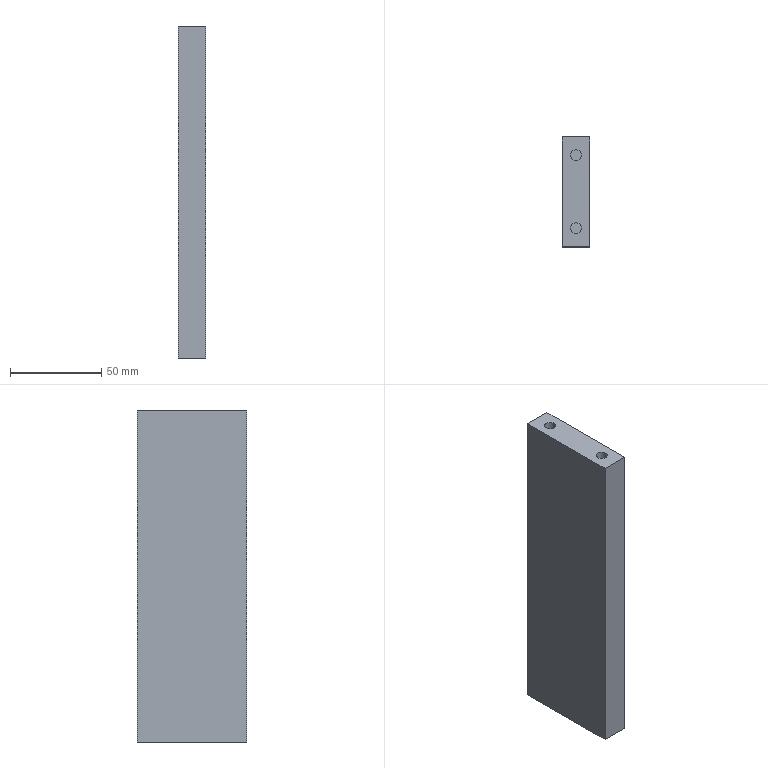Component | SolidWorks | CylinderSupportFrame02-1 | 1 solid | 18 faces | box 15 x 60 x 182 mm | volume 160973 mm3 | plane 10 | cylinder 8 | commonest cylinder face diameters 6 x8
build123d program:
from build123d import *

# Parameters (mm, degrees)
BOSS_EXTRUDE1_DEPTH                               = 60
SKETCH2_W                                         = 105
SKETCH2_H                                         = 15
BOSS_EXTRUDE2_DEPTH                               = 30
HOLE_SIZE_ACCORDING_TO_TYPE_OF_HEX_SO_D           = 6.6
HOLE_SIZE_ACCORDING_TO_TYPE_OF_HEX_SO_DEPTH       = 20
HOLE_SIZE_ACCORDING_TO_TYPE_OF_HEX_SO_CBORE_D     = 11
HOLE_SIZE_ACCORDING_TO_TYPE_OF_HEX_SO_CBORE_DEPTH = 6.8
LPATTERN1_COUNT                                   = 2
LPATTERN1_PITCH                                   = 30
SKETCH5_W                                         = 105
SKETCH5_H                                         = 15
SKETCH5_W_2                                       = 60
SKETCH5_H_2                                       = 20
CUT_EXTRUDE1_DEPTH                                = 279.727
M6_TAPPED_HOLE1_D                                 = 6
M6_TAPPED_HOLE1_DEPTH                             = 25


with BuildPart() as part:
    # Sketch1 → Boss-Extrude1 (new body)
    with BuildSketch(Plane(origin=(0, 0, 0), x_dir=(1, 0, 0), z_dir=(0, 1, 0))):
        Polygon((45, 0), (105, 0), (105, -20), (60, -20), (60, -202), (150, -202), (150, -217), (45, -217), align=None)
    extrude(amount=BOSS_EXTRUDE1_DEPTH)

    # Sketch2 → Boss-Extrude2 (add)
    with BuildSketch(Plane.XZ):
        with Locations((97.5, 209.5)):
            Rectangle(SKETCH2_W, SKETCH2_H)
    extrude(amount=BOSS_EXTRUDE2_DEPTH)

    # Hole Size _ according to_ type of Hex So
    with Locations(Plane(origin=(80, 15, 20), x_dir=(1, 0, 0), z_dir=(0, 0, 1))):
        with Locations((0, 0)):
            hole_size_according_to_type_of_hex_so = CounterBoreHole(HOLE_SIZE_ACCORDING_TO_TYPE_OF_HEX_SO_D / 2, HOLE_SIZE_ACCORDING_TO_TYPE_OF_HEX_SO_CBORE_D / 2, HOLE_SIZE_ACCORDING_TO_TYPE_OF_HEX_SO_CBORE_DEPTH, depth=HOLE_SIZE_ACCORDING_TO_TYPE_OF_HEX_SO_DEPTH)

    # LPattern1: Hole Size _ according to_ type of Hex So ×2
    with Locations(*[(0, i * LPATTERN1_PITCH, 0) for i in range(1, LPATTERN1_COUNT)]):
        add(hole_size_according_to_type_of_hex_so, mode=Mode.SUBTRACT)

    # Sketch5 → Cut-Extrude1 (cut, through all)
    with BuildSketch(Plane(origin=(0, 60, 0), x_dir=(1, 0, 0), z_dir=(0, 1, 0))):
        with Locations((97.5, -209.5)):
            Rectangle(SKETCH5_W, SKETCH5_H)
        with Locations((75, -10)):
            Rectangle(SKETCH5_W_2, SKETCH5_H_2)
    extrude(amount=-CUT_EXTRUDE1_DEPTH, mode=Mode.SUBTRACT)

    # M6 Tapped Hole1
    with Locations(Plane(origin=(52.5, 50, 20), x_dir=(-1, 0, 0), z_dir=(0, 0, -1))):
        with Locations((0, 0), (0, -40)):
            m6_tapped_hole1 = Hole(M6_TAPPED_HOLE1_D / 2, depth=M6_TAPPED_HOLE1_DEPTH)

    # Mirror1: M6 Tapped Hole1 across plane
    add(m6_tapped_hole1.mirror(Plane.XY.offset(111)), mode=Mode.SUBTRACT)


solid = part.part

# Placed as in the assembly
solid = solid.moved(Location((-44.66, -15.234, 38.104), (0, 0, 0)))
STEP:
#1=CARTESIAN_POINT('',(0.1906,1.369,8.469));
#2=VERTEX_POINT('',#1);
#3=CARTESIAN_POINT('',(0.4268,1.369,8.469));
#4=VERTEX_POINT('',#3);
#5=CARTESIAN_POINT('',(0.3087,1.369,8.469));
#6=DIRECTION('',(0.,0.,1.));
#7=DIRECTION('',(1.,0.,0.));
#8=AXIS2_PLACEMENT_3D('',#5,#6,#7);
#9=CIRCLE('',#8,0.1181);
#10=EDGE_CURVE('',#2,#4,#9,.T.);
#11=ORIENTED_EDGE('',*,*,#10,.F.);
#12=CARTESIAN_POINT('',(0.1906,1.369,9.453));
#13=VERTEX_POINT('',#12);
#14=CARTESIAN_POINT('',(0.1906,1.369,9.453));
#15=DIRECTION('',(0.,0.,1.));
#16=VECTOR('',#15,39.37);
#17=LINE('',#14,#16);
#18=EDGE_CURVE('',#2,#13,#17,.T.);
#19=ORIENTED_EDGE('',*,*,#18,.T.);
#20=CARTESIAN_POINT('',(0.4268,1.369,9.453));
#21=VERTEX_POINT('',#20);
#22=CARTESIAN_POINT('',(0.3087,1.369,9.453));
#23=DIRECTION('',(0.,0.,1.));
#24=DIRECTION('',(1.,0.,0.));
#25=AXIS2_PLACEMENT_3D('',#22,#23,#24);
#26=CIRCLE('',#25,0.1181);
#27=EDGE_CURVE('',#13,#21,#26,.T.);
#28=ORIENTED_EDGE('',*,*,#27,.T.);
#29=CARTESIAN_POINT('',(0.4268,1.369,9.453));
#30=DIRECTION('',(0.,0.,1.));
#31=VECTOR('',#30,39.37);
#32=LINE('',#29,#31);
#33=EDGE_CURVE('',#4,#21,#32,.T.);
#34=ORIENTED_EDGE('',*,*,#33,.F.);
#35=EDGE_LOOP('',(#11,#19,#28,#34));
#36=FACE_OUTER_BOUND('',#35,.T.);
#37=CARTESIAN_POINT('',(0.3087,1.369,9.453));
#38=DIRECTION('',(0.,0.,1.));
#39=DIRECTION('',(1.,0.,0.));
#40=AXIS2_PLACEMENT_3D('',#37,#38,#39);
#41=CYLINDRICAL_SURFACE('',#40,0.1181);
#42=ADVANCED_FACE('',(#36),#41,.F.);
#43=CARTESIAN_POINT('',(0.1906,-0.2061,8.469));
#44=VERTEX_POINT('',#43);
#45=CARTESIAN_POINT('',(0.4268,-0.2061,8.469));
#46=VERTEX_POINT('',#45);
#47=CARTESIAN_POINT('',(0.3087,-0.2061,8.469));
#48=DIRECTION('',(0.,0.,1.));
#49=DIRECTION('',(1.,0.,0.));
#50=AXIS2_PLACEMENT_3D('',#47,#48,#49);
#51=CIRCLE('',#50,0.1181);
#52=EDGE_CURVE('',#44,#46,#51,.T.);
#53=ORIENTED_EDGE('',*,*,#52,.F.);
#54=CARTESIAN_POINT('',(0.1906,-0.2061,9.453));
#55=VERTEX_POINT('',#54);
#56=CARTESIAN_POINT('',(0.1906,-0.2061,9.453));
#57=DIRECTION('',(0.,0.,1.));
#58=VECTOR('',#57,39.37);
#59=LINE('',#56,#58);
#60=EDGE_CURVE('',#44,#55,#59,.T.);
#61=ORIENTED_EDGE('',*,*,#60,.T.);
#62=CARTESIAN_POINT('',(0.4268,-0.2061,9.453));
#63=VERTEX_POINT('',#62);
#64=CARTESIAN_POINT('',(0.3087,-0.2061,9.453));
#65=DIRECTION('',(0.,0.,1.));
#66=DIRECTION('',(1.,0.,0.));
#67=AXIS2_PLACEMENT_3D('',#64,#65,#66);
#68=CIRCLE('',#67,0.1181);
#69=EDGE_CURVE('',#55,#63,#68,.T.);
#70=ORIENTED_EDGE('',*,*,#69,.T.);
#71=CARTESIAN_POINT('',(0.4268,-0.2061,9.453));
#72=DIRECTION('',(0.,0.,1.));
#73=VECTOR('',#72,39.37);
#74=LINE('',#71,#73);
#75=EDGE_CURVE('',#46,#63,#74,.T.);
#76=ORIENTED_EDGE('',*,*,#75,.F.);
#77=EDGE_LOOP('',(#53,#61,#70,#76));
#78=FACE_OUTER_BOUND('',#77,.T.);
#79=CARTESIAN_POINT('',(0.3087,-0.2061,9.453));
#80=DIRECTION('',(0.,0.,1.));
#81=DIRECTION('',(1.,0.,0.));
#82=AXIS2_PLACEMENT_3D('',#79,#80,#81);
#83=CYLINDRICAL_SURFACE('',#82,0.1181);
#84=ADVANCED_FACE('',(#78),#83,.F.);
#85=CARTESIAN_POINT('',(0.4268,1.369,3.272));
#86=VERTEX_POINT('',#85);
#87=CARTESIAN_POINT('',(0.1906,1.369,3.272));
#88=VERTEX_POINT('',#87);
#89=CARTESIAN_POINT('',(0.3087,1.369,3.272));
#90=DIRECTION('',(0.,0.,-1.));
#91=DIRECTION('',(-1.,0.,0.));
#92=AXIS2_PLACEMENT_3D('',#89,#90,#91);
#93=CIRCLE('',#92,0.1181);
#94=EDGE_CURVE('',#86,#88,#93,.T.);
#95=ORIENTED_EDGE('',*,*,#94,.F.);
#96=CARTESIAN_POINT('',(0.4268,1.369,2.288));
#97=VERTEX_POINT('',#96);
#98=CARTESIAN_POINT('',(0.4268,1.369,2.288));
#99=DIRECTION('',(0.,0.,-1.));
#100=VECTOR('',#99,39.37);
#101=LINE('',#98,#100);
#102=EDGE_CURVE('',#86,#97,#101,.T.);
#103=ORIENTED_EDGE('',*,*,#102,.T.);
#104=CARTESIAN_POINT('',(0.1906,1.369,2.288));
#105=VERTEX_POINT('',#104);
#106=CARTESIAN_POINT('',(0.3087,1.369,2.288));
#107=DIRECTION('',(0.,0.,-1.));
#108=DIRECTION('',(-1.,0.,0.));
#109=AXIS2_PLACEMENT_3D('',#106,#107,#108);
#110=CIRCLE('',#109,0.1181);
#111=EDGE_CURVE('',#97,#105,#110,.T.);
#112=ORIENTED_EDGE('',*,*,#111,.T.);
#113=CARTESIAN_POINT('',(0.1906,1.369,2.288));
#114=DIRECTION('',(0.,0.,-1.));
#115=VECTOR('',#114,39.37);
#116=LINE('',#113,#115);
#117=EDGE_CURVE('',#88,#105,#116,.T.);
#118=ORIENTED_EDGE('',*,*,#117,.F.);
#119=EDGE_LOOP('',(#95,#103,#112,#118));
#120=FACE_OUTER_BOUND('',#119,.T.);
#121=CARTESIAN_POINT('',(0.3087,1.369,2.288));
#122=DIRECTION('',(0.,0.,-1.));
#123=DIRECTION('',(-1.,0.,0.));
#124=AXIS2_PLACEMENT_3D('',#121,#122,#123);
#125=CYLINDRICAL_SURFACE('',#124,0.1181);
#126=ADVANCED_FACE('',(#120),#125,.F.);
#127=CARTESIAN_POINT('',(0.4268,-0.2061,3.272));
#128=VERTEX_POINT('',#127);
#129=CARTESIAN_POINT('',(0.1906,-0.2061,3.272));
#130=VERTEX_POINT('',#129);
#131=CARTESIAN_POINT('',(0.3087,-0.2061,3.272));
#132=DIRECTION('',(0.,0.,-1.));
#133=DIRECTION('',(-1.,0.,0.));
#134=AXIS2_PLACEMENT_3D('',#131,#132,#133);
#135=CIRCLE('',#134,0.1181);
#136=EDGE_CURVE('',#128,#130,#135,.T.);
#137=ORIENTED_EDGE('',*,*,#136,.F.);
#138=CARTESIAN_POINT('',(0.4268,-0.2061,2.288));
#139=VERTEX_POINT('',#138);
#140=CARTESIAN_POINT('',(0.4268,-0.2061,2.288));
#141=DIRECTION('',(0.,0.,-1.));
#142=VECTOR('',#141,39.37);
#143=LINE('',#140,#142);
#144=EDGE_CURVE('',#128,#139,#143,.T.);
#145=ORIENTED_EDGE('',*,*,#144,.T.);
#146=CARTESIAN_POINT('',(0.1906,-0.2061,2.288));
#147=VERTEX_POINT('',#146);
#148=CARTESIAN_POINT('',(0.3087,-0.2061,2.288));
#149=DIRECTION('',(0.,0.,-1.));
#150=DIRECTION('',(-1.,0.,0.));
#151=AXIS2_PLACEMENT_3D('',#148,#149,#150);
#152=CIRCLE('',#151,0.1181);
#153=EDGE_CURVE('',#139,#147,#152,.T.);
#154=ORIENTED_EDGE('',*,*,#153,.T.);
#155=CARTESIAN_POINT('',(0.1906,-0.2061,2.288));
#156=DIRECTION('',(0.,0.,-1.));
#157=VECTOR('',#156,39.37);
#158=LINE('',#155,#157);
#159=EDGE_CURVE('',#130,#147,#158,.T.);
#160=ORIENTED_EDGE('',*,*,#159,.F.);
#161=EDGE_LOOP('',(#137,#145,#154,#160));
#162=FACE_OUTER_BOUND('',#161,.T.);
#163=CARTESIAN_POINT('',(0.3087,-0.2061,2.288));
#164=DIRECTION('',(0.,0.,-1.));
#165=DIRECTION('',(-1.,0.,0.));
#166=AXIS2_PLACEMENT_3D('',#163,#164,#165);
#167=CYLINDRICAL_SURFACE('',#166,0.1181);
#168=ADVANCED_FACE('',(#162),#167,.F.);
#169=CARTESIAN_POINT('',(0.604,-0.5998,9.453));
#170=VERTEX_POINT('',#169);
#171=CARTESIAN_POINT('',(0.604,-0.5998,2.288));
#172=VERTEX_POINT('',#171);
#173=CARTESIAN_POINT('',(0.604,-0.5998,2.288));
#174=DIRECTION('',(-0.,0.,-1.));
#175=VECTOR('',#174,39.37);
#176=LINE('',#173,#175);
#177=EDGE_CURVE('',#170,#172,#176,.T.);
#178=ORIENTED_EDGE('',*,*,#177,.T.);
#179=CARTESIAN_POINT('',(0.604,1.762,2.288));
#180=VERTEX_POINT('',#179);
#181=CARTESIAN_POINT('',(0.604,1.762,2.288));
#182=DIRECTION('',(0.,-1.,0.));
#183=VECTOR('',#182,39.37);
#184=LINE('',#181,#183);
#185=EDGE_CURVE('',#180,#172,#184,.T.);
#186=ORIENTED_EDGE('',*,*,#185,.F.);
#187=CARTESIAN_POINT('',(0.604,1.762,9.453));
#188=VERTEX_POINT('',#187);
#189=CARTESIAN_POINT('',(0.604,1.762,2.288));
#190=DIRECTION('',(-0.,0.,-1.));
#191=VECTOR('',#190,39.37);
#192=LINE('',#189,#191);
#193=EDGE_CURVE('',#188,#180,#192,.T.);
#194=ORIENTED_EDGE('',*,*,#193,.F.);
#195=CARTESIAN_POINT('',(0.604,1.762,9.453));
#196=DIRECTION('',(0.,-1.,0.));
#197=VECTOR('',#196,39.37);
#198=LINE('',#195,#197);
#199=EDGE_CURVE('',#188,#170,#198,.T.);
#200=ORIENTED_EDGE('',*,*,#199,.T.);
#201=EDGE_LOOP('',(#178,#186,#194,#200));
#202=FACE_OUTER_BOUND('',#201,.T.);
#203=CARTESIAN_POINT('',(0.604,1.762,2.288));
#204=DIRECTION('',(-1.,0.,0.));
#205=DIRECTION('',(0.,0.,1.));
#206=AXIS2_PLACEMENT_3D('',#203,#204,#205);
#207=PLANE('',#206);
#208=ADVANCED_FACE('',(#202),#207,.F.);
#209=CARTESIAN_POINT('',(0.0134,-0.5998,2.288));
#210=VERTEX_POINT('',#209);
#211=CARTESIAN_POINT('',(0.0134,-0.5998,9.453));
#212=VERTEX_POINT('',#211);
#213=CARTESIAN_POINT('',(0.0134,-0.5998,1.5));
#214=DIRECTION('',(0.,0.,1.));
#215=VECTOR('',#214,39.37);
#216=LINE('',#213,#215);
#217=EDGE_CURVE('',#210,#212,#216,.T.);
#218=ORIENTED_EDGE('',*,*,#217,.T.);
#219=CARTESIAN_POINT('',(0.0134,1.762,9.453));
#220=VERTEX_POINT('',#219);
#221=CARTESIAN_POINT('',(0.0134,-1.781,9.453));
#222=DIRECTION('',(0.,1.,0.));
#223=VECTOR('',#222,39.37);
#224=LINE('',#221,#223);
#225=EDGE_CURVE('',#212,#220,#224,.T.);
#226=ORIENTED_EDGE('',*,*,#225,.T.);
#227=CARTESIAN_POINT('',(0.0134,1.762,2.288));
#228=VERTEX_POINT('',#227);
#229=CARTESIAN_POINT('',(0.0134,1.762,1.5));
#230=DIRECTION('',(0.,0.,1.));
#231=VECTOR('',#230,39.37);
#232=LINE('',#229,#231);
#233=EDGE_CURVE('',#228,#220,#232,.T.);
#234=ORIENTED_EDGE('',*,*,#233,.F.);
#235=CARTESIAN_POINT('',(0.0134,-1.781,2.288));
#236=DIRECTION('',(0.,1.,0.));
#237=VECTOR('',#236,39.37);
#238=LINE('',#235,#237);
#239=EDGE_CURVE('',#210,#228,#238,.T.);
#240=ORIENTED_EDGE('',*,*,#239,.F.);
#241=EDGE_LOOP('',(#218,#226,#234,#240));
#242=FACE_OUTER_BOUND('',#241,.T.);
#243=CARTESIAN_POINT('',(0.0134,1.762,1.5));
#244=DIRECTION('',(1.,0.,-0.));
#245=DIRECTION('',(-0.,0.,-1.));
#246=AXIS2_PLACEMENT_3D('',#243,#244,#245);
#247=PLANE('',#246);
#248=ADVANCED_FACE('',(#242),#247,.F.);
#249=ORIENTED_EDGE('',*,*,#233,.T.);
#250=CARTESIAN_POINT('',(0.0134,1.762,9.453));
#251=DIRECTION('',(-1.,0.,0.));
#252=VECTOR('',#251,39.37);
#253=LINE('',#250,#252);
#254=EDGE_CURVE('',#188,#220,#253,.T.);
#255=ORIENTED_EDGE('',*,*,#254,.F.);
#256=ORIENTED_EDGE('',*,*,#193,.T.);
#257=CARTESIAN_POINT('',(0.0134,1.762,2.288));
#258=DIRECTION('',(1.,0.,0.));
#259=VECTOR('',#258,39.37);
#260=LINE('',#257,#259);
#261=EDGE_CURVE('',#228,#180,#260,.T.);
#262=ORIENTED_EDGE('',*,*,#261,.F.);
#263=EDGE_LOOP('',(#249,#255,#256,#262));
#264=FACE_OUTER_BOUND('',#263,.T.);
#265=CARTESIAN_POINT('',(-1.758,1.762,1.5));
#266=DIRECTION('',(0.,-1.,0.));
#267=DIRECTION('',(0.,0.,-1.));
#268=AXIS2_PLACEMENT_3D('',#265,#266,#267);
#269=PLANE('',#268);
#270=ADVANCED_FACE('',(#264),#269,.F.);
#271=CARTESIAN_POINT('',(-1.758,-0.5998,2.288));
#272=DIRECTION('',(-1.,0.,0.));
#273=VECTOR('',#272,39.37);
#274=LINE('',#271,#273);
#275=EDGE_CURVE('',#172,#210,#274,.T.);
#276=ORIENTED_EDGE('',*,*,#275,.F.);
#277=ORIENTED_EDGE('',*,*,#177,.F.);
#278=CARTESIAN_POINT('',(4.147,-0.5998,9.453));
#279=DIRECTION('',(1.,0.,0.));
#280=VECTOR('',#279,39.37);
#281=LINE('',#278,#280);
#282=EDGE_CURVE('',#212,#170,#281,.T.);
#283=ORIENTED_EDGE('',*,*,#282,.F.);
#284=ORIENTED_EDGE('',*,*,#217,.F.);
#285=EDGE_LOOP('',(#276,#277,#283,#284));
#286=FACE_OUTER_BOUND('',#285,.T.);
#287=CARTESIAN_POINT('',(-1.758,-0.5998,1.5));
#288=DIRECTION('',(0.,-1.,0.));
#289=DIRECTION('',(0.,0.,-1.));
#290=AXIS2_PLACEMENT_3D('',#287,#288,#289);
#291=PLANE('',#290);
#292=ADVANCED_FACE('',(#286),#291,.T.);
#293=CARTESIAN_POINT('',(0.3087,1.369,2.288));
#294=DIRECTION('',(0.,0.,-1.));
#295=DIRECTION('',(-1.,0.,0.));
#296=AXIS2_PLACEMENT_3D('',#293,#294,#295);
#297=CIRCLE('',#296,0.1181);
#298=EDGE_CURVE('',#105,#97,#297,.T.);
#299=ORIENTED_EDGE('',*,*,#298,.F.);
#300=ORIENTED_EDGE('',*,*,#111,.F.);
#301=EDGE_LOOP('',(#299,#300));
#302=FACE_BOUND('',#301,.T.);
#303=CARTESIAN_POINT('',(0.3087,-0.2061,2.288));
#304=DIRECTION('',(0.,0.,-1.));
#305=DIRECTION('',(-1.,0.,0.));
#306=AXIS2_PLACEMENT_3D('',#303,#304,#305);
#307=CIRCLE('',#306,0.1181);
#308=EDGE_CURVE('',#147,#139,#307,.T.);
#309=ORIENTED_EDGE('',*,*,#308,.F.);
#310=ORIENTED_EDGE('',*,*,#153,.F.);
#311=EDGE_LOOP('',(#309,#310));
#312=FACE_BOUND('',#311,.T.);
#313=ORIENTED_EDGE('',*,*,#275,.T.);
#314=ORIENTED_EDGE('',*,*,#239,.T.);
#315=ORIENTED_EDGE('',*,*,#261,.T.);
#316=ORIENTED_EDGE('',*,*,#185,.T.);
#317=EDGE_LOOP('',(#313,#314,#315,#316));
#318=FACE_OUTER_BOUND('',#317,.T.);
#319=CARTESIAN_POINT('',(0.0134,-1.781,2.288));
#320=DIRECTION('',(0.,0.,1.));
#321=DIRECTION('',(1.,0.,0.));
#322=AXIS2_PLACEMENT_3D('',#319,#320,#321);
#323=PLANE('',#322);
#324=ADVANCED_FACE('',(#302,#312,#318),#323,.F.);
#325=CARTESIAN_POINT('',(0.3087,1.369,9.453));
#326=DIRECTION('',(0.,0.,1.));
#327=DIRECTION('',(1.,0.,0.));
#328=AXIS2_PLACEMENT_3D('',#325,#326,#327);
#329=CIRCLE('',#328,0.1181);
#330=EDGE_CURVE('',#21,#13,#329,.T.);
#331=ORIENTED_EDGE('',*,*,#330,.F.);
#332=ORIENTED_EDGE('',*,*,#27,.F.);
#333=EDGE_LOOP('',(#331,#332));
#334=FACE_BOUND('',#333,.T.);
#335=CARTESIAN_POINT('',(0.3087,-0.2061,9.453));
#336=DIRECTION('',(0.,0.,1.));
#337=DIRECTION('',(1.,0.,0.));
#338=AXIS2_PLACEMENT_3D('',#335,#336,#337);
#339=CIRCLE('',#338,0.1181);
#340=EDGE_CURVE('',#63,#55,#339,.T.);
#341=ORIENTED_EDGE('',*,*,#340,.F.);
#342=ORIENTED_EDGE('',*,*,#69,.F.);
#343=EDGE_LOOP('',(#341,#342));
#344=FACE_BOUND('',#343,.T.);
#345=ORIENTED_EDGE('',*,*,#254,.T.);
#346=ORIENTED_EDGE('',*,*,#225,.F.);
#347=ORIENTED_EDGE('',*,*,#282,.T.);
#348=ORIENTED_EDGE('',*,*,#199,.F.);
#349=EDGE_LOOP('',(#345,#346,#347,#348));
#350=FACE_OUTER_BOUND('',#349,.T.);
#351=CARTESIAN_POINT('',(0.0134,-1.781,9.453));
#352=DIRECTION('',(0.,0.,-1.));
#353=DIRECTION('',(-1.,0.,0.));
#354=AXIS2_PLACEMENT_3D('',#351,#352,#353);
#355=PLANE('',#354);
#356=ADVANCED_FACE('',(#334,#344,#350),#355,.F.);
#357=CARTESIAN_POINT('',(0.3087,-0.2061,3.272));
#358=DIRECTION('',(0.,0.,-1.));
#359=DIRECTION('',(-1.,0.,0.));
#360=AXIS2_PLACEMENT_3D('',#357,#358,#359);
#361=CIRCLE('',#360,0.1181);
#362=EDGE_CURVE('',#130,#128,#361,.T.);
#363=ORIENTED_EDGE('',*,*,#362,.T.);
#364=ORIENTED_EDGE('',*,*,#136,.T.);
#365=EDGE_LOOP('',(#363,#364));
#366=FACE_OUTER_BOUND('',#365,.T.);
#367=CARTESIAN_POINT('',(0.3087,-0.2061,3.272));
#368=DIRECTION('',(0.,0.,1.));
#369=DIRECTION('',(1.,0.,0.));
#370=AXIS2_PLACEMENT_3D('',#367,#368,#369);
#371=PLANE('',#370);
#372=ADVANCED_FACE('',(#366),#371,.F.);
#373=ORIENTED_EDGE('',*,*,#144,.F.);
#374=ORIENTED_EDGE('',*,*,#362,.F.);
#375=ORIENTED_EDGE('',*,*,#159,.T.);
#376=ORIENTED_EDGE('',*,*,#308,.T.);
#377=EDGE_LOOP('',(#373,#374,#375,#376));
#378=FACE_OUTER_BOUND('',#377,.T.);
#379=CARTESIAN_POINT('',(0.3087,-0.2061,2.288));
#380=DIRECTION('',(0.,0.,-1.));
#381=DIRECTION('',(-1.,0.,0.));
#382=AXIS2_PLACEMENT_3D('',#379,#380,#381);
#383=CYLINDRICAL_SURFACE('',#382,0.1181);
#384=ADVANCED_FACE('',(#378),#383,.F.);
#385=CARTESIAN_POINT('',(0.3087,1.369,3.272));
#386=DIRECTION('',(0.,0.,-1.));
#387=DIRECTION('',(-1.,0.,0.));
#388=AXIS2_PLACEMENT_3D('',#385,#386,#387);
#389=CIRCLE('',#388,0.1181);
#390=EDGE_CURVE('',#88,#86,#389,.T.);
#391=ORIENTED_EDGE('',*,*,#390,.T.);
#392=ORIENTED_EDGE('',*,*,#94,.T.);
#393=EDGE_LOOP('',(#391,#392));
#394=FACE_OUTER_BOUND('',#393,.T.);
#395=CARTESIAN_POINT('',(0.3087,1.369,3.272));
#396=DIRECTION('',(0.,0.,1.));
#397=DIRECTION('',(1.,0.,0.));
#398=AXIS2_PLACEMENT_3D('',#395,#396,#397);
#399=PLANE('',#398);
#400=ADVANCED_FACE('',(#394),#399,.F.);
#401=ORIENTED_EDGE('',*,*,#102,.F.);
#402=ORIENTED_EDGE('',*,*,#390,.F.);
#403=ORIENTED_EDGE('',*,*,#117,.T.);
#404=ORIENTED_EDGE('',*,*,#298,.T.);
#405=EDGE_LOOP('',(#401,#402,#403,#404));
#406=FACE_OUTER_BOUND('',#405,.T.);
#407=CARTESIAN_POINT('',(0.3087,1.369,2.288));
#408=DIRECTION('',(0.,0.,-1.));
#409=DIRECTION('',(-1.,0.,0.));
#410=AXIS2_PLACEMENT_3D('',#407,#408,#409);
#411=CYLINDRICAL_SURFACE('',#410,0.1181);
#412=ADVANCED_FACE('',(#406),#411,.F.);
#413=CARTESIAN_POINT('',(0.3087,-0.2061,8.469));
#414=DIRECTION('',(0.,0.,1.));
#415=DIRECTION('',(1.,0.,0.));
#416=AXIS2_PLACEMENT_3D('',#413,#414,#415);
#417=CIRCLE('',#416,0.1181);
#418=EDGE_CURVE('',#46,#44,#417,.T.);
#419=ORIENTED_EDGE('',*,*,#418,.T.);
#420=ORIENTED_EDGE('',*,*,#52,.T.);
#421=EDGE_LOOP('',(#419,#420));
#422=FACE_OUTER_BOUND('',#421,.T.);
#423=CARTESIAN_POINT('',(0.3087,-0.2061,8.469));
#424=DIRECTION('',(0.,0.,-1.));
#425=DIRECTION('',(-1.,0.,0.));
#426=AXIS2_PLACEMENT_3D('',#423,#424,#425);
#427=PLANE('',#426);
#428=ADVANCED_FACE('',(#422),#427,.F.);
#429=ORIENTED_EDGE('',*,*,#60,.F.);
#430=ORIENTED_EDGE('',*,*,#418,.F.);
#431=ORIENTED_EDGE('',*,*,#75,.T.);
#432=ORIENTED_EDGE('',*,*,#340,.T.);
#433=EDGE_LOOP('',(#429,#430,#431,#432));
#434=FACE_OUTER_BOUND('',#433,.T.);
#435=CARTESIAN_POINT('',(0.3087,-0.2061,9.453));
#436=DIRECTION('',(0.,0.,1.));
#437=DIRECTION('',(1.,0.,0.));
#438=AXIS2_PLACEMENT_3D('',#435,#436,#437);
#439=CYLINDRICAL_SURFACE('',#438,0.1181);
#440=ADVANCED_FACE('',(#434),#439,.F.);
#441=CARTESIAN_POINT('',(0.3087,1.369,8.469));
#442=DIRECTION('',(0.,0.,1.));
#443=DIRECTION('',(1.,0.,0.));
#444=AXIS2_PLACEMENT_3D('',#441,#442,#443);
#445=CIRCLE('',#444,0.1181);
#446=EDGE_CURVE('',#4,#2,#445,.T.);
#447=ORIENTED_EDGE('',*,*,#446,.T.);
#448=ORIENTED_EDGE('',*,*,#10,.T.);
#449=EDGE_LOOP('',(#447,#448));
#450=FACE_OUTER_BOUND('',#449,.T.);
#451=CARTESIAN_POINT('',(0.3087,1.369,8.469));
#452=DIRECTION('',(0.,0.,-1.));
#453=DIRECTION('',(-1.,0.,0.));
#454=AXIS2_PLACEMENT_3D('',#451,#452,#453);
#455=PLANE('',#454);
#456=ADVANCED_FACE('',(#450),#455,.F.);
#457=ORIENTED_EDGE('',*,*,#18,.F.);
#458=ORIENTED_EDGE('',*,*,#446,.F.);
#459=ORIENTED_EDGE('',*,*,#33,.T.);
#460=ORIENTED_EDGE('',*,*,#330,.T.);
#461=EDGE_LOOP('',(#457,#458,#459,#460));
#462=FACE_OUTER_BOUND('',#461,.T.);
#463=CARTESIAN_POINT('',(0.3087,1.369,9.453));
#464=DIRECTION('',(0.,0.,1.));
#465=DIRECTION('',(1.,0.,0.));
#466=AXIS2_PLACEMENT_3D('',#463,#464,#465);
#467=CYLINDRICAL_SURFACE('',#466,0.1181);
#468=ADVANCED_FACE('',(#462),#467,.F.);
#469=CLOSED_SHELL('',(#42,#84,#126,#168,#208,#248,#270,#292,#324,#356,#372,#384,#400,#412,#428,#440,#456,#468));
#470=MANIFOLD_SOLID_BREP('',#469);
#471=CARTESIAN_POINT('',(0.,0.,0.));
#472=DIRECTION('',(0.,0.,1.));
#473=DIRECTION('',(1.,0.,0.));
#474=AXIS2_PLACEMENT_3D('',#471,#472,#473);
#475=(LENGTH_UNIT()NAMED_UNIT(*)SI_UNIT($,.METRE.));
#476=LENGTH_MEASURE_WITH_UNIT(LENGTH_MEASURE(0.0254),#475);
#477=DIMENSIONAL_EXPONENTS(1.,0.,0.,0.,0.,0.,0.);
#478=(CONVERSION_BASED_UNIT('',#476)LENGTH_UNIT()NAMED_UNIT(#477));
#479=UNCERTAINTY_MEASURE_WITH_UNIT(LENGTH_MEASURE(0.00001),#478,'','');
#480=(NAMED_UNIT(*)PLANE_ANGLE_UNIT()SI_UNIT($,.RADIAN.));
#481=(NAMED_UNIT(*)SI_UNIT($,.STERADIAN.)SOLID_ANGLE_UNIT());
#482=(GEOMETRIC_REPRESENTATION_CONTEXT(3)GLOBAL_UNCERTAINTY_ASSIGNED_CONTEXT((#479))GLOBAL_UNIT_ASSIGNED_CONTEXT((#478,#480,#481))REPRESENTATION_CONTEXT('',''));
#483=ADVANCED_BREP_SHAPE_REPRESENTATION('',(#470,#474),#482);
#484=COLOUR_RGB('',0.7922,0.8196,0.9333);
#485=FILL_AREA_STYLE_COLOUR('',#484);
#486=FILL_AREA_STYLE('',(#485));
#487=SURFACE_STYLE_FILL_AREA(#486);
#488=SURFACE_SIDE_STYLE('',(#487));
#489=SURFACE_STYLE_USAGE(.BOTH.,#488);
#490=PRESENTATION_STYLE_ASSIGNMENT((#489));
#491=STYLED_ITEM('',(#490),#470);
#492=PRESENTATION_LAYER_ASSIGNMENT('','',(#491));
#493=(LENGTH_UNIT()NAMED_UNIT(*)SI_UNIT($,.METRE.));
#494=LENGTH_MEASURE_WITH_UNIT(LENGTH_MEASURE(0.0254),#493);
#495=DIMENSIONAL_EXPONENTS(1.,0.,0.,0.,0.,0.,0.);
#496=(CONVERSION_BASED_UNIT('',#494)LENGTH_UNIT()NAMED_UNIT(#495));
#497=UNCERTAINTY_MEASURE_WITH_UNIT(LENGTH_MEASURE(0.00001),#496,'','');
#498=(NAMED_UNIT(*)PLANE_ANGLE_UNIT()SI_UNIT($,.RADIAN.));
#499=(NAMED_UNIT(*)SI_UNIT($,.STERADIAN.)SOLID_ANGLE_UNIT());
#500=(GEOMETRIC_REPRESENTATION_CONTEXT(3)GLOBAL_UNCERTAINTY_ASSIGNED_CONTEXT((#497))GLOBAL_UNIT_ASSIGNED_CONTEXT((#496,#498,#499))REPRESENTATION_CONTEXT('',''));
#501=MECHANICAL_DESIGN_GEOMETRIC_PRESENTATION_REPRESENTATION('',(#491),#500);